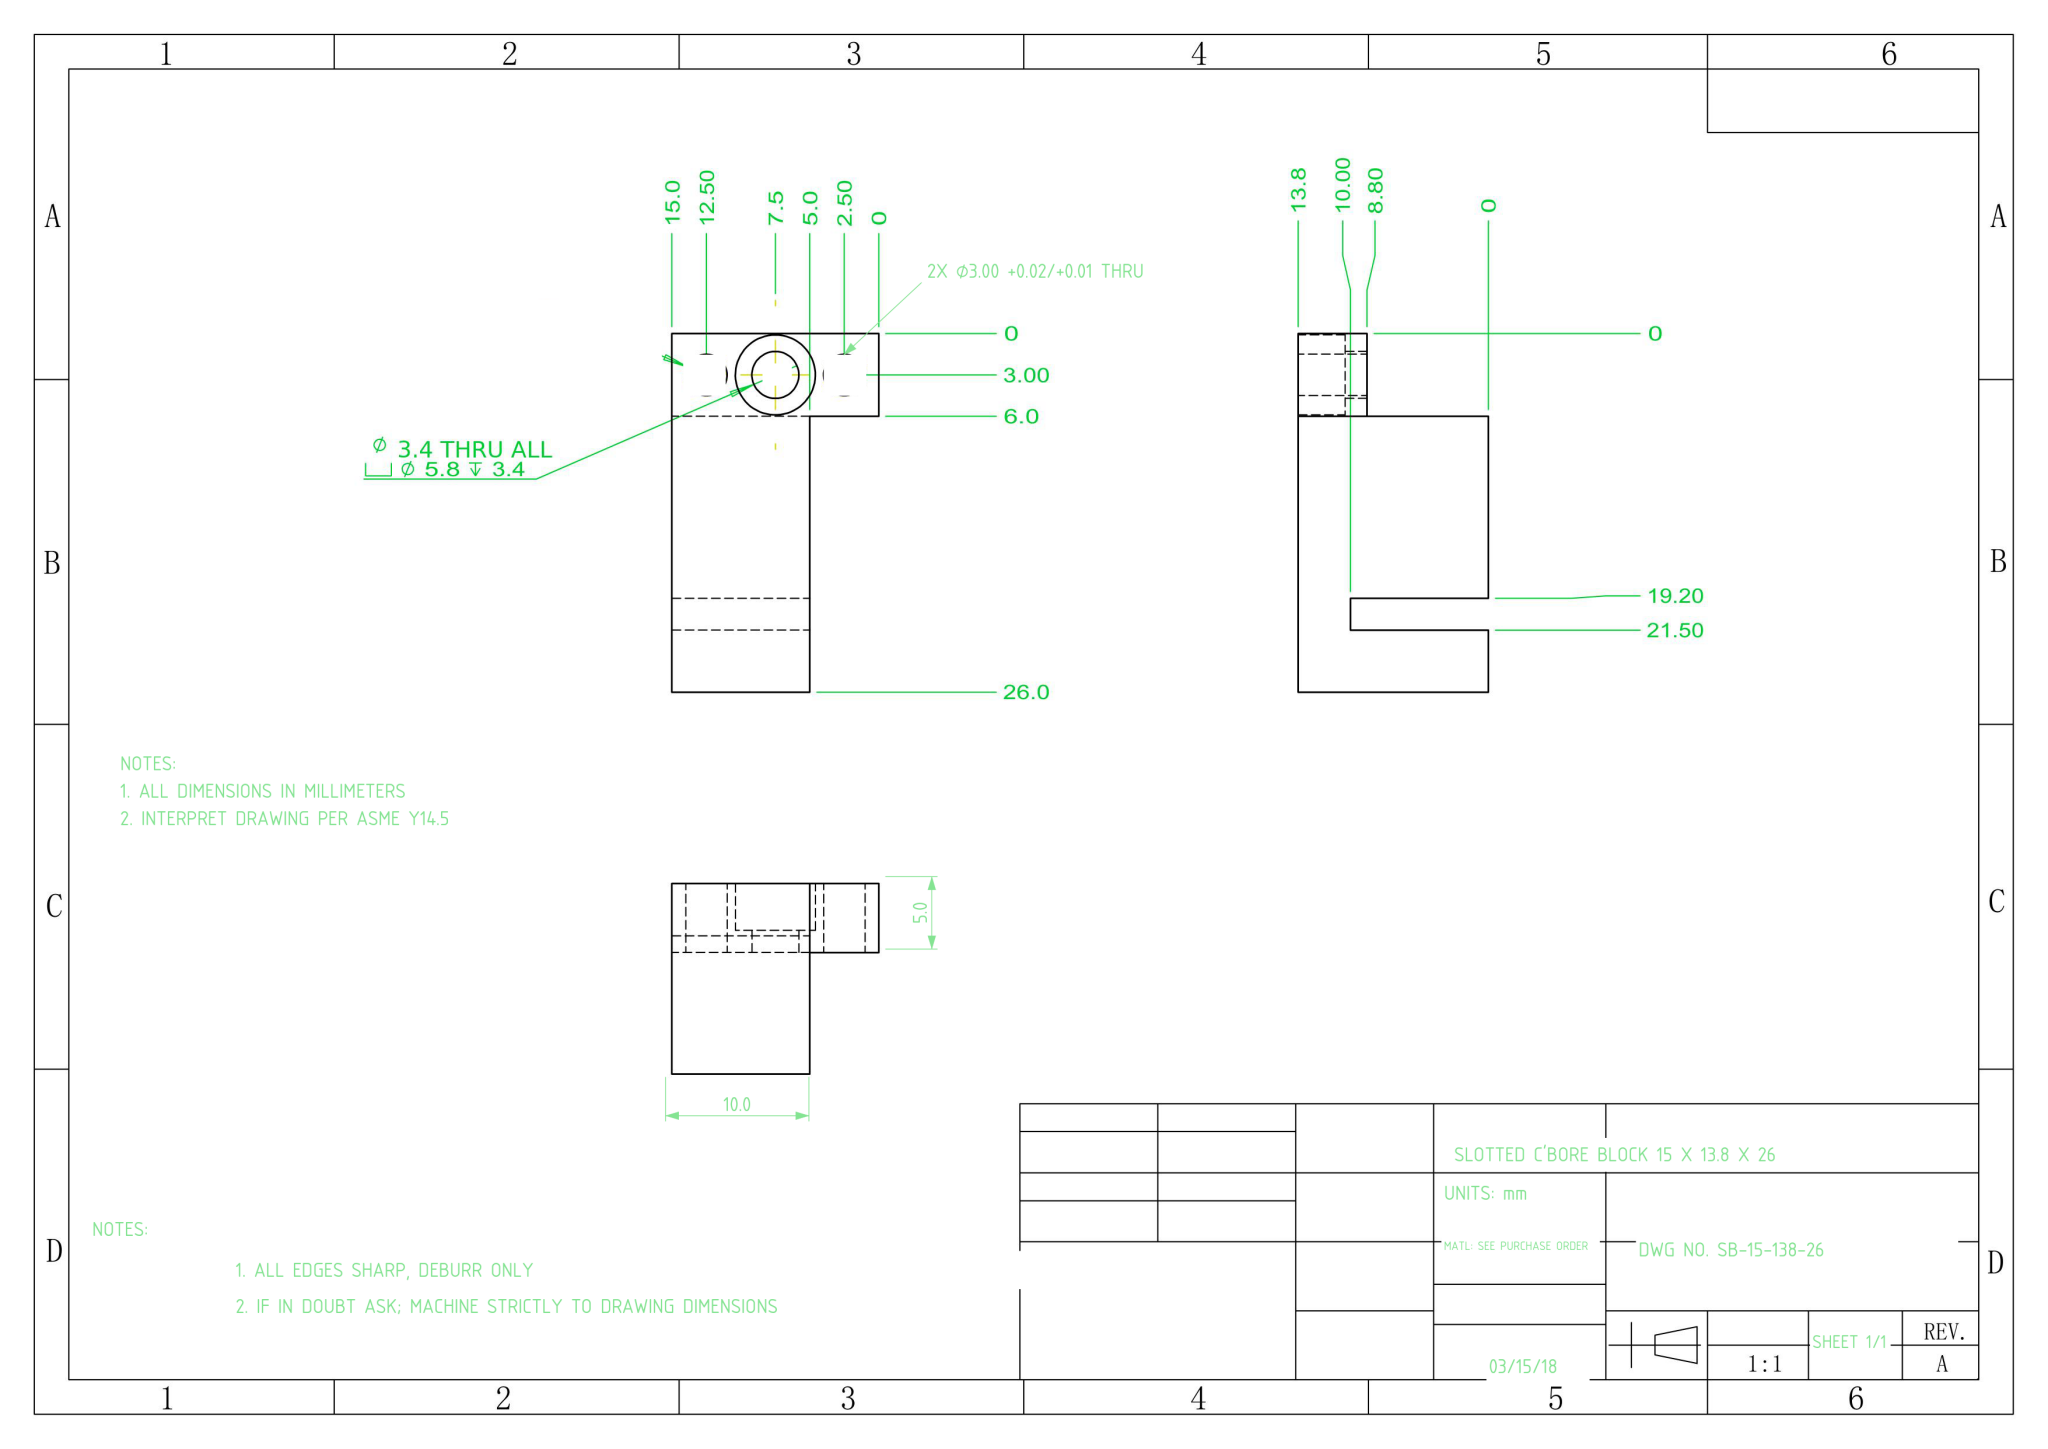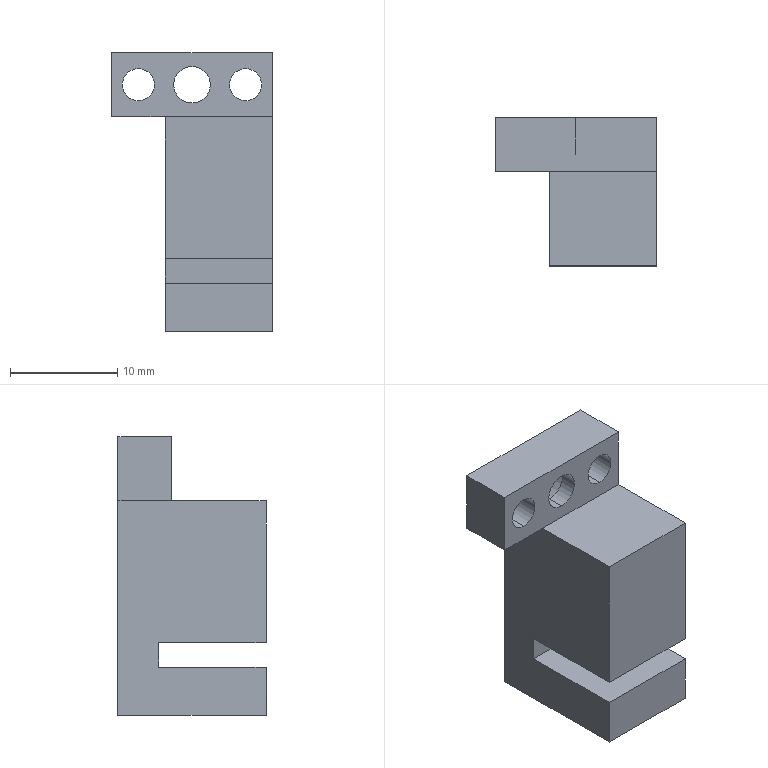Part | NX | mm | 1 solid | 23 faces | box 15 x 13.8 x 26 mm | volume 2805 mm3 | plane 15 | cylinder 8 | commonest cylinder face diameters 3 x4 5.8 x2 3.4 x2
STEP:
#1=COLOUR_RGB('',1.,0.4039,0.4431);
#2=FILL_AREA_STYLE_COLOUR('',#1);
#3=FILL_AREA_STYLE('',(#2));
#4=SURFACE_STYLE_FILL_AREA(#3);
#5=SURFACE_SIDE_STYLE('',(#4));
#6=SURFACE_STYLE_USAGE(.BOTH.,#5);
#7=PRESENTATION_STYLE_ASSIGNMENT((#6));
#8=CARTESIAN_POINT('',(2.5,-3.4,20.1));
#9=VERTEX_POINT('',#8);
#10=CARTESIAN_POINT('',(2.5,-3.4,25.9));
#11=VERTEX_POINT('',#10);
#12=CARTESIAN_POINT('',(2.5,-3.4,23.));
#13=DIRECTION('',(0.,1.,0.));
#14=DIRECTION('',(0.,0.,1.));
#15=AXIS2_PLACEMENT_3D('',#12,#13,#14);
#16=CIRCLE('',#15,2.9);
#17=EDGE_CURVE('',#9,#11,#16,.T.);
#18=ORIENTED_EDGE('',*,*,#17,.F.);
#19=CARTESIAN_POINT('',(2.5,0.,20.1));
#20=VERTEX_POINT('',#19);
#21=CARTESIAN_POINT('',(2.5,0.,20.1));
#22=DIRECTION('',(0.,1.,0.));
#23=VECTOR('',#22,1000.);
#24=LINE('',#21,#23);
#25=EDGE_CURVE('',#9,#20,#24,.T.);
#26=ORIENTED_EDGE('',*,*,#25,.T.);
#27=CARTESIAN_POINT('',(2.5,0.,25.9));
#28=VERTEX_POINT('',#27);
#29=CARTESIAN_POINT('',(2.5,0.,23.));
#30=DIRECTION('',(0.,1.,0.));
#31=DIRECTION('',(0.,0.,1.));
#32=AXIS2_PLACEMENT_3D('',#29,#30,#31);
#33=CIRCLE('',#32,2.9);
#34=EDGE_CURVE('',#20,#28,#33,.T.);
#35=ORIENTED_EDGE('',*,*,#34,.T.);
#36=CARTESIAN_POINT('',(2.5,0.,25.9));
#37=DIRECTION('',(0.,1.,0.));
#38=VECTOR('',#37,1000.);
#39=LINE('',#36,#38);
#40=EDGE_CURVE('',#11,#28,#39,.T.);
#41=ORIENTED_EDGE('',*,*,#40,.F.);
#42=EDGE_LOOP('',(#18,#26,#35,#41));
#43=FACE_OUTER_BOUND('',#42,.T.);
#44=CARTESIAN_POINT('',(2.5,0.,23.));
#45=DIRECTION('',(0.,1.,0.));
#46=DIRECTION('',(0.,0.,1.));
#47=AXIS2_PLACEMENT_3D('',#44,#45,#46);
#48=CYLINDRICAL_SURFACE('',#47,2.9);
#49=ADVANCED_FACE('',(#43),#48,.F.);
#50=CARTESIAN_POINT('',(2.5,-5.,21.3));
#51=VERTEX_POINT('',#50);
#52=CARTESIAN_POINT('',(2.5,-5.,24.7));
#53=VERTEX_POINT('',#52);
#54=CARTESIAN_POINT('',(2.5,-5.,23.));
#55=DIRECTION('',(0.,1.,0.));
#56=DIRECTION('',(0.,0.,1.));
#57=AXIS2_PLACEMENT_3D('',#54,#55,#56);
#58=CIRCLE('',#57,1.7);
#59=EDGE_CURVE('',#51,#53,#58,.T.);
#60=ORIENTED_EDGE('',*,*,#59,.F.);
#61=CARTESIAN_POINT('',(2.5,-3.4,21.3));
#62=VERTEX_POINT('',#61);
#63=CARTESIAN_POINT('',(2.5,0.,21.3));
#64=DIRECTION('',(0.,1.,0.));
#65=VECTOR('',#64,1000.);
#66=LINE('',#63,#65);
#67=EDGE_CURVE('',#51,#62,#66,.T.);
#68=ORIENTED_EDGE('',*,*,#67,.T.);
#69=CARTESIAN_POINT('',(2.5,-3.4,24.7));
#70=VERTEX_POINT('',#69);
#71=CARTESIAN_POINT('',(2.5,-3.4,23.));
#72=DIRECTION('',(0.,1.,0.));
#73=DIRECTION('',(0.,0.,1.));
#74=AXIS2_PLACEMENT_3D('',#71,#72,#73);
#75=CIRCLE('',#74,1.7);
#76=EDGE_CURVE('',#62,#70,#75,.T.);
#77=ORIENTED_EDGE('',*,*,#76,.T.);
#78=CARTESIAN_POINT('',(2.5,0.,24.7));
#79=DIRECTION('',(0.,1.,0.));
#80=VECTOR('',#79,1000.);
#81=LINE('',#78,#80);
#82=EDGE_CURVE('',#53,#70,#81,.T.);
#83=ORIENTED_EDGE('',*,*,#82,.F.);
#84=EDGE_LOOP('',(#60,#68,#77,#83));
#85=FACE_OUTER_BOUND('',#84,.T.);
#86=CARTESIAN_POINT('',(2.5,0.,23.));
#87=DIRECTION('',(0.,1.,0.));
#88=DIRECTION('',(0.,0.,1.));
#89=AXIS2_PLACEMENT_3D('',#86,#87,#88);
#90=CYLINDRICAL_SURFACE('',#89,1.7);
#91=ADVANCED_FACE('',(#85),#90,.F.);
#92=CARTESIAN_POINT('',(7.5,-5.,21.5));
#93=VERTEX_POINT('',#92);
#94=CARTESIAN_POINT('',(7.5,-5.,24.5));
#95=VERTEX_POINT('',#94);
#96=CARTESIAN_POINT('',(7.5,-5.,23.));
#97=DIRECTION('',(0.,1.,0.));
#98=DIRECTION('',(0.,0.,1.));
#99=AXIS2_PLACEMENT_3D('',#96,#97,#98);
#100=CIRCLE('',#99,1.5);
#101=EDGE_CURVE('',#93,#95,#100,.T.);
#102=ORIENTED_EDGE('',*,*,#101,.F.);
#103=CARTESIAN_POINT('',(7.5,0.,21.5));
#104=VERTEX_POINT('',#103);
#105=CARTESIAN_POINT('',(7.5,0.,21.5));
#106=DIRECTION('',(0.,1.,0.));
#107=VECTOR('',#106,1000.);
#108=LINE('',#105,#107);
#109=EDGE_CURVE('',#93,#104,#108,.T.);
#110=ORIENTED_EDGE('',*,*,#109,.T.);
#111=CARTESIAN_POINT('',(7.5,0.,24.5));
#112=VERTEX_POINT('',#111);
#113=CARTESIAN_POINT('',(7.5,0.,23.));
#114=DIRECTION('',(0.,1.,0.));
#115=DIRECTION('',(0.,0.,1.));
#116=AXIS2_PLACEMENT_3D('',#113,#114,#115);
#117=CIRCLE('',#116,1.5);
#118=EDGE_CURVE('',#104,#112,#117,.T.);
#119=ORIENTED_EDGE('',*,*,#118,.T.);
#120=CARTESIAN_POINT('',(7.5,0.,24.5));
#121=DIRECTION('',(0.,1.,0.));
#122=VECTOR('',#121,1000.);
#123=LINE('',#120,#122);
#124=EDGE_CURVE('',#95,#112,#123,.T.);
#125=ORIENTED_EDGE('',*,*,#124,.F.);
#126=EDGE_LOOP('',(#102,#110,#119,#125));
#127=FACE_OUTER_BOUND('',#126,.T.);
#128=CARTESIAN_POINT('',(7.5,0.,23.));
#129=DIRECTION('',(0.,1.,0.));
#130=DIRECTION('',(0.,0.,1.));
#131=AXIS2_PLACEMENT_3D('',#128,#129,#130);
#132=CYLINDRICAL_SURFACE('',#131,1.5);
#133=ADVANCED_FACE('',(#127),#132,.F.);
#134=CARTESIAN_POINT('',(-2.5,-5.,21.5));
#135=VERTEX_POINT('',#134);
#136=CARTESIAN_POINT('',(-2.5,-5.,24.5));
#137=VERTEX_POINT('',#136);
#138=CARTESIAN_POINT('',(-2.5,-5.,23.));
#139=DIRECTION('',(0.,1.,0.));
#140=DIRECTION('',(0.,0.,1.));
#141=AXIS2_PLACEMENT_3D('',#138,#139,#140);
#142=CIRCLE('',#141,1.5);
#143=EDGE_CURVE('',#135,#137,#142,.T.);
#144=ORIENTED_EDGE('',*,*,#143,.F.);
#145=CARTESIAN_POINT('',(-2.5,0.,21.5));
#146=VERTEX_POINT('',#145);
#147=CARTESIAN_POINT('',(-2.5,0.,21.5));
#148=DIRECTION('',(0.,1.,0.));
#149=VECTOR('',#148,1000.);
#150=LINE('',#147,#149);
#151=EDGE_CURVE('',#135,#146,#150,.T.);
#152=ORIENTED_EDGE('',*,*,#151,.T.);
#153=CARTESIAN_POINT('',(-2.5,0.,24.5));
#154=VERTEX_POINT('',#153);
#155=CARTESIAN_POINT('',(-2.5,0.,23.));
#156=DIRECTION('',(0.,1.,0.));
#157=DIRECTION('',(0.,0.,1.));
#158=AXIS2_PLACEMENT_3D('',#155,#156,#157);
#159=CIRCLE('',#158,1.5);
#160=EDGE_CURVE('',#146,#154,#159,.T.);
#161=ORIENTED_EDGE('',*,*,#160,.T.);
#162=CARTESIAN_POINT('',(-2.5,0.,24.5));
#163=DIRECTION('',(0.,1.,0.));
#164=VECTOR('',#163,1000.);
#165=LINE('',#162,#164);
#166=EDGE_CURVE('',#137,#154,#165,.T.);
#167=ORIENTED_EDGE('',*,*,#166,.F.);
#168=EDGE_LOOP('',(#144,#152,#161,#167));
#169=FACE_OUTER_BOUND('',#168,.T.);
#170=CARTESIAN_POINT('',(-2.5,0.,23.));
#171=DIRECTION('',(0.,1.,0.));
#172=DIRECTION('',(0.,0.,1.));
#173=AXIS2_PLACEMENT_3D('',#170,#171,#172);
#174=CYLINDRICAL_SURFACE('',#173,1.5);
#175=ADVANCED_FACE('',(#169),#174,.F.);
#176=CARTESIAN_POINT('',(10.,-13.8,4.5));
#177=VERTEX_POINT('',#176);
#178=CARTESIAN_POINT('',(10.,-13.8,0.));
#179=VERTEX_POINT('',#178);
#180=CARTESIAN_POINT('',(10.,-13.8,20.));
#181=DIRECTION('',(0.,0.,-1.));
#182=VECTOR('',#181,1000.);
#183=LINE('',#180,#182);
#184=EDGE_CURVE('',#177,#179,#183,.T.);
#185=ORIENTED_EDGE('',*,*,#184,.F.);
#186=CARTESIAN_POINT('',(0.,-13.8,4.5));
#187=VERTEX_POINT('',#186);
#188=CARTESIAN_POINT('',(10.,-13.8,4.5));
#189=DIRECTION('',(-1.,-0.,0.));
#190=VECTOR('',#189,1000.);
#191=LINE('',#188,#190);
#192=EDGE_CURVE('',#177,#187,#191,.T.);
#193=ORIENTED_EDGE('',*,*,#192,.T.);
#194=CARTESIAN_POINT('',(0.,-13.8,0.));
#195=VERTEX_POINT('',#194);
#196=CARTESIAN_POINT('',(0.,-13.8,20.));
#197=DIRECTION('',(0.,0.,-1.));
#198=VECTOR('',#197,1000.);
#199=LINE('',#196,#198);
#200=EDGE_CURVE('',#187,#195,#199,.T.);
#201=ORIENTED_EDGE('',*,*,#200,.T.);
#202=CARTESIAN_POINT('',(0.,-13.8,0.));
#203=DIRECTION('',(1.,0.,0.));
#204=VECTOR('',#203,1000.);
#205=LINE('',#202,#204);
#206=EDGE_CURVE('',#195,#179,#205,.T.);
#207=ORIENTED_EDGE('',*,*,#206,.T.);
#208=EDGE_LOOP('',(#185,#193,#201,#207));
#209=FACE_OUTER_BOUND('',#208,.T.);
#210=CARTESIAN_POINT('',(0.,-13.8,20.));
#211=DIRECTION('',(0.,1.,0.));
#212=DIRECTION('',(0.,0.,1.));
#213=AXIS2_PLACEMENT_3D('',#210,#211,#212);
#214=PLANE('',#213);
#215=ADVANCED_FACE('',(#209),#214,.F.);
#216=ORIENTED_EDGE('',*,*,#200,.F.);
#217=CARTESIAN_POINT('',(0.,-3.8,4.5));
#218=VERTEX_POINT('',#217);
#219=CARTESIAN_POINT('',(0.,-13.8,4.5));
#220=DIRECTION('',(0.,-1.,0.));
#221=VECTOR('',#220,1000.);
#222=LINE('',#219,#221);
#223=EDGE_CURVE('',#218,#187,#222,.T.);
#224=ORIENTED_EDGE('',*,*,#223,.F.);
#225=CARTESIAN_POINT('',(0.,-3.8,6.8));
#226=VERTEX_POINT('',#225);
#227=CARTESIAN_POINT('',(0.,-3.8,4.5));
#228=DIRECTION('',(0.,0.,-1.));
#229=VECTOR('',#228,1000.);
#230=LINE('',#227,#229);
#231=EDGE_CURVE('',#226,#218,#230,.T.);
#232=ORIENTED_EDGE('',*,*,#231,.F.);
#233=CARTESIAN_POINT('',(0.,-13.8,6.8));
#234=VERTEX_POINT('',#233);
#235=CARTESIAN_POINT('',(0.,-13.8,6.8));
#236=DIRECTION('',(-0.,1.,0.));
#237=VECTOR('',#236,1000.);
#238=LINE('',#235,#237);
#239=EDGE_CURVE('',#234,#226,#238,.T.);
#240=ORIENTED_EDGE('',*,*,#239,.F.);
#241=CARTESIAN_POINT('',(0.,-13.8,20.));
#242=VERTEX_POINT('',#241);
#243=CARTESIAN_POINT('',(0.,-13.8,20.));
#244=DIRECTION('',(0.,0.,-1.));
#245=VECTOR('',#244,1000.);
#246=LINE('',#243,#245);
#247=EDGE_CURVE('',#242,#234,#246,.T.);
#248=ORIENTED_EDGE('',*,*,#247,.F.);
#249=CARTESIAN_POINT('',(0.,-5.,20.));
#250=VERTEX_POINT('',#249);
#251=CARTESIAN_POINT('',(0.,0.,20.));
#252=DIRECTION('',(0.,-1.,0.));
#253=VECTOR('',#252,1000.);
#254=LINE('',#251,#253);
#255=EDGE_CURVE('',#250,#242,#254,.T.);
#256=ORIENTED_EDGE('',*,*,#255,.F.);
#257=CARTESIAN_POINT('',(0.,0.,20.));
#258=VERTEX_POINT('',#257);
#259=CARTESIAN_POINT('',(0.,0.,20.));
#260=DIRECTION('',(0.,-1.,0.));
#261=VECTOR('',#260,1000.);
#262=LINE('',#259,#261);
#263=EDGE_CURVE('',#258,#250,#262,.T.);
#264=ORIENTED_EDGE('',*,*,#263,.F.);
#265=CARTESIAN_POINT('',(0.,0.,0.));
#266=VERTEX_POINT('',#265);
#267=CARTESIAN_POINT('',(0.,0.,20.));
#268=DIRECTION('',(0.,0.,-1.));
#269=VECTOR('',#268,1000.);
#270=LINE('',#267,#269);
#271=EDGE_CURVE('',#258,#266,#270,.T.);
#272=ORIENTED_EDGE('',*,*,#271,.T.);
#273=CARTESIAN_POINT('',(0.,0.,0.));
#274=DIRECTION('',(0.,-1.,0.));
#275=VECTOR('',#274,1000.);
#276=LINE('',#273,#275);
#277=EDGE_CURVE('',#266,#195,#276,.T.);
#278=ORIENTED_EDGE('',*,*,#277,.T.);
#279=EDGE_LOOP('',(#216,#224,#232,#240,#248,#256,#264,#272,#278));
#280=FACE_OUTER_BOUND('',#279,.T.);
#281=CARTESIAN_POINT('',(0.,0.,20.));
#282=DIRECTION('',(1.,0.,0.));
#283=DIRECTION('',(-0.,1.,0.));
#284=AXIS2_PLACEMENT_3D('',#281,#282,#283);
#285=PLANE('',#284);
#286=ADVANCED_FACE('',(#280),#285,.F.);
#287=ORIENTED_EDGE('',*,*,#247,.T.);
#288=CARTESIAN_POINT('',(10.,-13.8,6.8));
#289=VERTEX_POINT('',#288);
#290=CARTESIAN_POINT('',(10.,-13.8,6.8));
#291=DIRECTION('',(-1.,-0.,0.));
#292=VECTOR('',#291,1000.);
#293=LINE('',#290,#292);
#294=EDGE_CURVE('',#289,#234,#293,.T.);
#295=ORIENTED_EDGE('',*,*,#294,.F.);
#296=CARTESIAN_POINT('',(10.,-13.8,20.));
#297=VERTEX_POINT('',#296);
#298=CARTESIAN_POINT('',(10.,-13.8,20.));
#299=DIRECTION('',(0.,0.,-1.));
#300=VECTOR('',#299,1000.);
#301=LINE('',#298,#300);
#302=EDGE_CURVE('',#297,#289,#301,.T.);
#303=ORIENTED_EDGE('',*,*,#302,.F.);
#304=CARTESIAN_POINT('',(0.,-13.8,20.));
#305=DIRECTION('',(1.,0.,0.));
#306=VECTOR('',#305,1000.);
#307=LINE('',#304,#306);
#308=EDGE_CURVE('',#242,#297,#307,.T.);
#309=ORIENTED_EDGE('',*,*,#308,.F.);
#310=EDGE_LOOP('',(#287,#295,#303,#309));
#311=FACE_OUTER_BOUND('',#310,.T.);
#312=CARTESIAN_POINT('',(0.,-13.8,20.));
#313=DIRECTION('',(0.,1.,0.));
#314=DIRECTION('',(0.,0.,1.));
#315=AXIS2_PLACEMENT_3D('',#312,#313,#314);
#316=PLANE('',#315);
#317=ADVANCED_FACE('',(#311),#316,.F.);
#318=CARTESIAN_POINT('',(10.,-3.8,6.8));
#319=VERTEX_POINT('',#318);
#320=CARTESIAN_POINT('',(10.,-3.8,4.5));
#321=VERTEX_POINT('',#320);
#322=CARTESIAN_POINT('',(10.,-3.8,4.5));
#323=DIRECTION('',(0.,0.,-1.));
#324=VECTOR('',#323,1000.);
#325=LINE('',#322,#324);
#326=EDGE_CURVE('',#319,#321,#325,.T.);
#327=ORIENTED_EDGE('',*,*,#326,.T.);
#328=CARTESIAN_POINT('',(10.,-13.8,4.5));
#329=DIRECTION('',(0.,-1.,0.));
#330=VECTOR('',#329,1000.);
#331=LINE('',#328,#330);
#332=EDGE_CURVE('',#321,#177,#331,.T.);
#333=ORIENTED_EDGE('',*,*,#332,.T.);
#334=ORIENTED_EDGE('',*,*,#184,.T.);
#335=CARTESIAN_POINT('',(10.,0.,0.));
#336=VERTEX_POINT('',#335);
#337=CARTESIAN_POINT('',(10.,0.,0.));
#338=DIRECTION('',(-0.,1.,0.));
#339=VECTOR('',#338,1000.);
#340=LINE('',#337,#339);
#341=EDGE_CURVE('',#179,#336,#340,.T.);
#342=ORIENTED_EDGE('',*,*,#341,.T.);
#343=CARTESIAN_POINT('',(10.,0.,26.));
#344=VERTEX_POINT('',#343);
#345=CARTESIAN_POINT('',(10.,0.,20.));
#346=DIRECTION('',(0.,0.,-1.));
#347=VECTOR('',#346,1000.);
#348=LINE('',#345,#347);
#349=EDGE_CURVE('',#344,#336,#348,.T.);
#350=ORIENTED_EDGE('',*,*,#349,.F.);
#351=CARTESIAN_POINT('',(10.,-5.,26.));
#352=VERTEX_POINT('',#351);
#353=CARTESIAN_POINT('',(10.,0.,26.));
#354=DIRECTION('',(0.,1.,0.));
#355=VECTOR('',#354,1000.);
#356=LINE('',#353,#355);
#357=EDGE_CURVE('',#352,#344,#356,.T.);
#358=ORIENTED_EDGE('',*,*,#357,.F.);
#359=CARTESIAN_POINT('',(10.,-5.,20.));
#360=VERTEX_POINT('',#359);
#361=CARTESIAN_POINT('',(10.,-5.,26.));
#362=DIRECTION('',(0.,0.,-1.));
#363=VECTOR('',#362,1000.);
#364=LINE('',#361,#363);
#365=EDGE_CURVE('',#352,#360,#364,.T.);
#366=ORIENTED_EDGE('',*,*,#365,.T.);
#367=CARTESIAN_POINT('',(10.,0.,20.));
#368=DIRECTION('',(-0.,1.,0.));
#369=VECTOR('',#368,1000.);
#370=LINE('',#367,#369);
#371=EDGE_CURVE('',#297,#360,#370,.T.);
#372=ORIENTED_EDGE('',*,*,#371,.F.);
#373=ORIENTED_EDGE('',*,*,#302,.T.);
#374=CARTESIAN_POINT('',(10.,-13.8,6.8));
#375=DIRECTION('',(-0.,1.,0.));
#376=VECTOR('',#375,1000.);
#377=LINE('',#374,#376);
#378=EDGE_CURVE('',#289,#319,#377,.T.);
#379=ORIENTED_EDGE('',*,*,#378,.T.);
#380=EDGE_LOOP('',(#327,#333,#334,#342,#350,#358,#366,#372,#373,#379));
#381=FACE_OUTER_BOUND('',#380,.T.);
#382=CARTESIAN_POINT('',(10.,0.,20.));
#383=DIRECTION('',(-1.,-0.,0.));
#384=DIRECTION('',(0.,-1.,0.));
#385=AXIS2_PLACEMENT_3D('',#382,#383,#384);
#386=PLANE('',#385);
#387=ADVANCED_FACE('',(#381),#386,.F.);
#388=CARTESIAN_POINT('',(2.5,0.,23.));
#389=DIRECTION('',(0.,1.,0.));
#390=DIRECTION('',(0.,0.,1.));
#391=AXIS2_PLACEMENT_3D('',#388,#389,#390);
#392=CIRCLE('',#391,2.9);
#393=EDGE_CURVE('',#28,#20,#392,.T.);
#394=ORIENTED_EDGE('',*,*,#393,.F.);
#395=ORIENTED_EDGE('',*,*,#34,.F.);
#396=EDGE_LOOP('',(#394,#395));
#397=FACE_BOUND('',#396,.T.);
#398=CARTESIAN_POINT('',(7.5,0.,23.));
#399=DIRECTION('',(0.,1.,0.));
#400=DIRECTION('',(0.,0.,1.));
#401=AXIS2_PLACEMENT_3D('',#398,#399,#400);
#402=CIRCLE('',#401,1.5);
#403=EDGE_CURVE('',#112,#104,#402,.T.);
#404=ORIENTED_EDGE('',*,*,#403,.F.);
#405=ORIENTED_EDGE('',*,*,#118,.F.);
#406=EDGE_LOOP('',(#404,#405));
#407=FACE_BOUND('',#406,.T.);
#408=CARTESIAN_POINT('',(-2.5,0.,23.));
#409=DIRECTION('',(0.,1.,0.));
#410=DIRECTION('',(0.,0.,1.));
#411=AXIS2_PLACEMENT_3D('',#408,#409,#410);
#412=CIRCLE('',#411,1.5);
#413=EDGE_CURVE('',#154,#146,#412,.T.);
#414=ORIENTED_EDGE('',*,*,#413,.F.);
#415=ORIENTED_EDGE('',*,*,#160,.F.);
#416=EDGE_LOOP('',(#414,#415));
#417=FACE_BOUND('',#416,.T.);
#418=CARTESIAN_POINT('',(0.,0.,0.));
#419=DIRECTION('',(-1.,0.,0.));
#420=VECTOR('',#419,1000.);
#421=LINE('',#418,#420);
#422=EDGE_CURVE('',#336,#266,#421,.T.);
#423=ORIENTED_EDGE('',*,*,#422,.T.);
#424=ORIENTED_EDGE('',*,*,#271,.F.);
#425=CARTESIAN_POINT('',(-5.,-0.,20.));
#426=VERTEX_POINT('',#425);
#427=CARTESIAN_POINT('',(-5.,-0.,20.));
#428=DIRECTION('',(1.,0.,0.));
#429=VECTOR('',#428,1000.);
#430=LINE('',#427,#429);
#431=EDGE_CURVE('',#426,#258,#430,.T.);
#432=ORIENTED_EDGE('',*,*,#431,.F.);
#433=CARTESIAN_POINT('',(-5.,0.,26.));
#434=VERTEX_POINT('',#433);
#435=CARTESIAN_POINT('',(-5.,0.,26.));
#436=DIRECTION('',(0.,-0.,-1.));
#437=VECTOR('',#436,1000.);
#438=LINE('',#435,#437);
#439=EDGE_CURVE('',#434,#426,#438,.T.);
#440=ORIENTED_EDGE('',*,*,#439,.F.);
#441=CARTESIAN_POINT('',(0.,0.,26.));
#442=DIRECTION('',(-1.,0.,0.));
#443=VECTOR('',#442,1000.);
#444=LINE('',#441,#443);
#445=EDGE_CURVE('',#344,#434,#444,.T.);
#446=ORIENTED_EDGE('',*,*,#445,.F.);
#447=ORIENTED_EDGE('',*,*,#349,.T.);
#448=EDGE_LOOP('',(#423,#424,#432,#440,#446,#447));
#449=FACE_OUTER_BOUND('',#448,.T.);
#450=CARTESIAN_POINT('',(0.,0.,20.));
#451=DIRECTION('',(0.,-1.,0.));
#452=DIRECTION('',(0.,0.,-1.));
#453=AXIS2_PLACEMENT_3D('',#450,#451,#452);
#454=PLANE('',#453);
#455=ADVANCED_FACE('',(#397,#407,#417,#449),#454,.F.);
#456=CARTESIAN_POINT('',(0.,-5.,20.));
#457=DIRECTION('',(1.,0.,0.));
#458=VECTOR('',#457,1000.);
#459=LINE('',#456,#458);
#460=EDGE_CURVE('',#250,#360,#459,.T.);
#461=ORIENTED_EDGE('',*,*,#460,.F.);
#462=ORIENTED_EDGE('',*,*,#255,.T.);
#463=ORIENTED_EDGE('',*,*,#308,.T.);
#464=ORIENTED_EDGE('',*,*,#371,.T.);
#465=EDGE_LOOP('',(#461,#462,#463,#464));
#466=FACE_OUTER_BOUND('',#465,.T.);
#467=CARTESIAN_POINT('',(0.,0.,20.));
#468=DIRECTION('',(0.,0.,1.));
#469=DIRECTION('',(1.,0.,0.));
#470=AXIS2_PLACEMENT_3D('',#467,#468,#469);
#471=PLANE('',#470);
#472=ADVANCED_FACE('',(#466),#471,.T.);
#473=ORIENTED_EDGE('',*,*,#277,.F.);
#474=ORIENTED_EDGE('',*,*,#422,.F.);
#475=ORIENTED_EDGE('',*,*,#341,.F.);
#476=ORIENTED_EDGE('',*,*,#206,.F.);
#477=EDGE_LOOP('',(#473,#474,#475,#476));
#478=FACE_OUTER_BOUND('',#477,.T.);
#479=CARTESIAN_POINT('',(0.,0.,0.));
#480=DIRECTION('',(0.,0.,1.));
#481=DIRECTION('',(1.,0.,0.));
#482=AXIS2_PLACEMENT_3D('',#479,#480,#481);
#483=PLANE('',#482);
#484=ADVANCED_FACE('',(#478),#483,.F.);
#485=CARTESIAN_POINT('',(2.5,-5.,23.));
#486=DIRECTION('',(0.,1.,0.));
#487=DIRECTION('',(0.,0.,1.));
#488=AXIS2_PLACEMENT_3D('',#485,#486,#487);
#489=CIRCLE('',#488,1.7);
#490=EDGE_CURVE('',#53,#51,#489,.T.);
#491=ORIENTED_EDGE('',*,*,#490,.T.);
#492=ORIENTED_EDGE('',*,*,#59,.T.);
#493=EDGE_LOOP('',(#491,#492));
#494=FACE_BOUND('',#493,.T.);
#495=CARTESIAN_POINT('',(7.5,-5.,23.));
#496=DIRECTION('',(0.,1.,0.));
#497=DIRECTION('',(0.,0.,1.));
#498=AXIS2_PLACEMENT_3D('',#495,#496,#497);
#499=CIRCLE('',#498,1.5);
#500=EDGE_CURVE('',#95,#93,#499,.T.);
#501=ORIENTED_EDGE('',*,*,#500,.T.);
#502=ORIENTED_EDGE('',*,*,#101,.T.);
#503=EDGE_LOOP('',(#501,#502));
#504=FACE_BOUND('',#503,.T.);
#505=CARTESIAN_POINT('',(-2.5,-5.,23.));
#506=DIRECTION('',(0.,1.,0.));
#507=DIRECTION('',(0.,0.,1.));
#508=AXIS2_PLACEMENT_3D('',#505,#506,#507);
#509=CIRCLE('',#508,1.5);
#510=EDGE_CURVE('',#137,#135,#509,.T.);
#511=ORIENTED_EDGE('',*,*,#510,.T.);
#512=ORIENTED_EDGE('',*,*,#143,.T.);
#513=EDGE_LOOP('',(#511,#512));
#514=FACE_BOUND('',#513,.T.);
#515=ORIENTED_EDGE('',*,*,#460,.T.);
#516=ORIENTED_EDGE('',*,*,#365,.F.);
#517=CARTESIAN_POINT('',(-5.,-5.,26.));
#518=VERTEX_POINT('',#517);
#519=CARTESIAN_POINT('',(0.,-5.,26.));
#520=DIRECTION('',(1.,0.,0.));
#521=VECTOR('',#520,1000.);
#522=LINE('',#519,#521);
#523=EDGE_CURVE('',#518,#352,#522,.T.);
#524=ORIENTED_EDGE('',*,*,#523,.F.);
#525=CARTESIAN_POINT('',(-5.,-5.,20.));
#526=VERTEX_POINT('',#525);
#527=CARTESIAN_POINT('',(-5.,-5.,26.));
#528=DIRECTION('',(-0.,0.,1.));
#529=VECTOR('',#528,1000.);
#530=LINE('',#527,#529);
#531=EDGE_CURVE('',#526,#518,#530,.T.);
#532=ORIENTED_EDGE('',*,*,#531,.F.);
#533=CARTESIAN_POINT('',(-5.,-5.,20.));
#534=DIRECTION('',(1.,0.,0.));
#535=VECTOR('',#534,1000.);
#536=LINE('',#533,#535);
#537=EDGE_CURVE('',#526,#250,#536,.T.);
#538=ORIENTED_EDGE('',*,*,#537,.T.);
#539=EDGE_LOOP('',(#515,#516,#524,#532,#538));
#540=FACE_OUTER_BOUND('',#539,.T.);
#541=CARTESIAN_POINT('',(0.,-5.,26.));
#542=DIRECTION('',(0.,1.,0.));
#543=DIRECTION('',(0.,0.,1.));
#544=AXIS2_PLACEMENT_3D('',#541,#542,#543);
#545=PLANE('',#544);
#546=ADVANCED_FACE('',(#494,#504,#514,#540),#545,.F.);
#547=ORIENTED_EDGE('',*,*,#445,.T.);
#548=CARTESIAN_POINT('',(-5.,0.,26.));
#549=DIRECTION('',(-0.,1.,0.));
#550=VECTOR('',#549,1000.);
#551=LINE('',#548,#550);
#552=EDGE_CURVE('',#518,#434,#551,.T.);
#553=ORIENTED_EDGE('',*,*,#552,.F.);
#554=ORIENTED_EDGE('',*,*,#523,.T.);
#555=ORIENTED_EDGE('',*,*,#357,.T.);
#556=EDGE_LOOP('',(#547,#553,#554,#555));
#557=FACE_OUTER_BOUND('',#556,.T.);
#558=CARTESIAN_POINT('',(0.,0.,26.));
#559=DIRECTION('',(0.,0.,1.));
#560=DIRECTION('',(1.,0.,0.));
#561=AXIS2_PLACEMENT_3D('',#558,#559,#560);
#562=PLANE('',#561);
#563=ADVANCED_FACE('',(#557),#562,.T.);
#564=ORIENTED_EDGE('',*,*,#263,.T.);
#565=ORIENTED_EDGE('',*,*,#537,.F.);
#566=CARTESIAN_POINT('',(-5.,-0.,20.));
#567=DIRECTION('',(0.,-1.,0.));
#568=VECTOR('',#567,1000.);
#569=LINE('',#566,#568);
#570=EDGE_CURVE('',#426,#526,#569,.T.);
#571=ORIENTED_EDGE('',*,*,#570,.F.);
#572=ORIENTED_EDGE('',*,*,#431,.T.);
#573=EDGE_LOOP('',(#564,#565,#571,#572));
#574=FACE_OUTER_BOUND('',#573,.T.);
#575=CARTESIAN_POINT('',(-5.,-0.,20.));
#576=DIRECTION('',(0.,0.,1.));
#577=DIRECTION('',(1.,0.,0.));
#578=AXIS2_PLACEMENT_3D('',#575,#576,#577);
#579=PLANE('',#578);
#580=ADVANCED_FACE('',(#574),#579,.F.);
#581=ORIENTED_EDGE('',*,*,#552,.T.);
#582=ORIENTED_EDGE('',*,*,#439,.T.);
#583=ORIENTED_EDGE('',*,*,#570,.T.);
#584=ORIENTED_EDGE('',*,*,#531,.T.);
#585=EDGE_LOOP('',(#581,#582,#583,#584));
#586=FACE_OUTER_BOUND('',#585,.T.);
#587=CARTESIAN_POINT('',(-5.,-0.,0.));
#588=DIRECTION('',(1.,0.,-0.));
#589=DIRECTION('',(-0.,1.,0.));
#590=AXIS2_PLACEMENT_3D('',#587,#588,#589);
#591=PLANE('',#590);
#592=ADVANCED_FACE('',(#586),#591,.F.);
#593=ORIENTED_EDGE('',*,*,#223,.T.);
#594=ORIENTED_EDGE('',*,*,#192,.F.);
#595=ORIENTED_EDGE('',*,*,#332,.F.);
#596=CARTESIAN_POINT('',(10.,-3.8,4.5));
#597=DIRECTION('',(-1.,-0.,0.));
#598=VECTOR('',#597,1000.);
#599=LINE('',#596,#598);
#600=EDGE_CURVE('',#321,#218,#599,.T.);
#601=ORIENTED_EDGE('',*,*,#600,.T.);
#602=EDGE_LOOP('',(#593,#594,#595,#601));
#603=FACE_OUTER_BOUND('',#602,.T.);
#604=CARTESIAN_POINT('',(10.,-13.8,4.5));
#605=DIRECTION('',(0.,-0.,-1.));
#606=DIRECTION('',(0.,1.,-0.));
#607=AXIS2_PLACEMENT_3D('',#604,#605,#606);
#608=PLANE('',#607);
#609=ADVANCED_FACE('',(#603),#608,.F.);
#610=ORIENTED_EDGE('',*,*,#231,.T.);
#611=ORIENTED_EDGE('',*,*,#600,.F.);
#612=ORIENTED_EDGE('',*,*,#326,.F.);
#613=CARTESIAN_POINT('',(10.,-3.8,6.8));
#614=DIRECTION('',(-1.,-0.,0.));
#615=VECTOR('',#614,1000.);
#616=LINE('',#613,#615);
#617=EDGE_CURVE('',#319,#226,#616,.T.);
#618=ORIENTED_EDGE('',*,*,#617,.T.);
#619=EDGE_LOOP('',(#610,#611,#612,#618));
#620=FACE_OUTER_BOUND('',#619,.T.);
#621=CARTESIAN_POINT('',(10.,-3.8,4.5));
#622=DIRECTION('',(-0.,1.,0.));
#623=DIRECTION('',(-1.,-0.,0.));
#624=AXIS2_PLACEMENT_3D('',#621,#622,#623);
#625=PLANE('',#624);
#626=ADVANCED_FACE('',(#620),#625,.F.);
#627=ORIENTED_EDGE('',*,*,#239,.T.);
#628=ORIENTED_EDGE('',*,*,#617,.F.);
#629=ORIENTED_EDGE('',*,*,#378,.F.);
#630=ORIENTED_EDGE('',*,*,#294,.T.);
#631=EDGE_LOOP('',(#627,#628,#629,#630));
#632=FACE_OUTER_BOUND('',#631,.T.);
#633=CARTESIAN_POINT('',(10.,-13.8,6.8));
#634=DIRECTION('',(0.,0.,1.));
#635=DIRECTION('',(1.,0.,0.));
#636=AXIS2_PLACEMENT_3D('',#633,#634,#635);
#637=PLANE('',#636);
#638=ADVANCED_FACE('',(#632),#637,.F.);
#639=ORIENTED_EDGE('',*,*,#151,.F.);
#640=ORIENTED_EDGE('',*,*,#510,.F.);
#641=ORIENTED_EDGE('',*,*,#166,.T.);
#642=ORIENTED_EDGE('',*,*,#413,.T.);
#643=EDGE_LOOP('',(#639,#640,#641,#642));
#644=FACE_OUTER_BOUND('',#643,.T.);
#645=CARTESIAN_POINT('',(-2.5,0.,23.));
#646=DIRECTION('',(0.,1.,0.));
#647=DIRECTION('',(0.,0.,1.));
#648=AXIS2_PLACEMENT_3D('',#645,#646,#647);
#649=CYLINDRICAL_SURFACE('',#648,1.5);
#650=ADVANCED_FACE('',(#644),#649,.F.);
#651=ORIENTED_EDGE('',*,*,#109,.F.);
#652=ORIENTED_EDGE('',*,*,#500,.F.);
#653=ORIENTED_EDGE('',*,*,#124,.T.);
#654=ORIENTED_EDGE('',*,*,#403,.T.);
#655=EDGE_LOOP('',(#651,#652,#653,#654));
#656=FACE_OUTER_BOUND('',#655,.T.);
#657=CARTESIAN_POINT('',(7.5,0.,23.));
#658=DIRECTION('',(0.,1.,0.));
#659=DIRECTION('',(0.,0.,1.));
#660=AXIS2_PLACEMENT_3D('',#657,#658,#659);
#661=CYLINDRICAL_SURFACE('',#660,1.5);
#662=ADVANCED_FACE('',(#656),#661,.F.);
#663=ORIENTED_EDGE('',*,*,#67,.F.);
#664=ORIENTED_EDGE('',*,*,#490,.F.);
#665=ORIENTED_EDGE('',*,*,#82,.T.);
#666=CARTESIAN_POINT('',(2.5,-3.4,23.));
#667=DIRECTION('',(0.,1.,0.));
#668=DIRECTION('',(0.,0.,1.));
#669=AXIS2_PLACEMENT_3D('',#666,#667,#668);
#670=CIRCLE('',#669,1.7);
#671=EDGE_CURVE('',#70,#62,#670,.T.);
#672=ORIENTED_EDGE('',*,*,#671,.T.);
#673=EDGE_LOOP('',(#663,#664,#665,#672));
#674=FACE_OUTER_BOUND('',#673,.T.);
#675=CARTESIAN_POINT('',(2.5,0.,23.));
#676=DIRECTION('',(0.,1.,0.));
#677=DIRECTION('',(0.,0.,1.));
#678=AXIS2_PLACEMENT_3D('',#675,#676,#677);
#679=CYLINDRICAL_SURFACE('',#678,1.7);
#680=ADVANCED_FACE('',(#674),#679,.F.);
#681=ORIENTED_EDGE('',*,*,#671,.F.);
#682=ORIENTED_EDGE('',*,*,#76,.F.);
#683=EDGE_LOOP('',(#681,#682));
#684=FACE_BOUND('',#683,.T.);
#685=CARTESIAN_POINT('',(2.5,-3.4,23.));
#686=DIRECTION('',(0.,1.,0.));
#687=DIRECTION('',(0.,0.,1.));
#688=AXIS2_PLACEMENT_3D('',#685,#686,#687);
#689=CIRCLE('',#688,2.9);
#690=EDGE_CURVE('',#11,#9,#689,.T.);
#691=ORIENTED_EDGE('',*,*,#690,.T.);
#692=ORIENTED_EDGE('',*,*,#17,.T.);
#693=EDGE_LOOP('',(#691,#692));
#694=FACE_OUTER_BOUND('',#693,.T.);
#695=CARTESIAN_POINT('',(4.2,-3.4,23.));
#696=DIRECTION('',(0.,-1.,0.));
#697=DIRECTION('',(0.,0.,-1.));
#698=AXIS2_PLACEMENT_3D('',#695,#696,#697);
#699=PLANE('',#698);
#700=ADVANCED_FACE('',(#684,#694),#699,.F.);
#701=ORIENTED_EDGE('',*,*,#25,.F.);
#702=ORIENTED_EDGE('',*,*,#690,.F.);
#703=ORIENTED_EDGE('',*,*,#40,.T.);
#704=ORIENTED_EDGE('',*,*,#393,.T.);
#705=EDGE_LOOP('',(#701,#702,#703,#704));
#706=FACE_OUTER_BOUND('',#705,.T.);
#707=CARTESIAN_POINT('',(2.5,0.,23.));
#708=DIRECTION('',(0.,1.,0.));
#709=DIRECTION('',(0.,0.,1.));
#710=AXIS2_PLACEMENT_3D('',#707,#708,#709);
#711=CYLINDRICAL_SURFACE('',#710,2.9);
#712=ADVANCED_FACE('',(#706),#711,.F.);
#713=CLOSED_SHELL('',(#49,#91,#133,#175,#215,#286,#317,#387,#455,#472,#484,#546,#563,#580,#592,#609,#626,#638,#650,#662,#680,#700,#712));
#714=MANIFOLD_SOLID_BREP('',#713);
#715=CARTESIAN_POINT('',(0.,0.,0.));
#716=DIRECTION('',(0.,0.,1.));
#717=DIRECTION('',(1.,0.,0.));
#718=AXIS2_PLACEMENT_3D('',#715,#716,#717);
#719=(LENGTH_UNIT()NAMED_UNIT(*)SI_UNIT(.MILLI.,.METRE.));
#720=UNCERTAINTY_MEASURE_WITH_UNIT(LENGTH_MEASURE(0.00001),#719,'','');
#721=(NAMED_UNIT(*)PLANE_ANGLE_UNIT()SI_UNIT($,.RADIAN.));
#722=(NAMED_UNIT(*)SI_UNIT($,.STERADIAN.)SOLID_ANGLE_UNIT());
#723=(GEOMETRIC_REPRESENTATION_CONTEXT(3)GLOBAL_UNCERTAINTY_ASSIGNED_CONTEXT((#720))GLOBAL_UNIT_ASSIGNED_CONTEXT((#719,#721,#722))REPRESENTATION_CONTEXT('',''));
#724=ADVANCED_BREP_SHAPE_REPRESENTATION('',(#714,#718),#723);
#725=STYLED_ITEM('',(#7),#724);
#726=PRESENTATION_LAYER_ASSIGNMENT('','',(#725));
#727=COLOUR_RGB('',1.,0.4039,0.4431);
#728=FILL_AREA_STYLE_COLOUR('',#727);
#729=FILL_AREA_STYLE('',(#728));
#730=SURFACE_STYLE_FILL_AREA(#729);
#731=SURFACE_SIDE_STYLE('',(#730));
#732=SURFACE_STYLE_USAGE(.BOTH.,#731);
#733=PRESENTATION_STYLE_ASSIGNMENT((#732));
#734=STYLED_ITEM('',(#733),#714);
#735=(LENGTH_UNIT()NAMED_UNIT(*)SI_UNIT(.MILLI.,.METRE.));
#736=UNCERTAINTY_MEASURE_WITH_UNIT(LENGTH_MEASURE(0.00001),#735,'','');
#737=(NAMED_UNIT(*)PLANE_ANGLE_UNIT()SI_UNIT($,.RADIAN.));
#738=(NAMED_UNIT(*)SI_UNIT($,.STERADIAN.)SOLID_ANGLE_UNIT());
#739=(GEOMETRIC_REPRESENTATION_CONTEXT(3)GLOBAL_UNCERTAINTY_ASSIGNED_CONTEXT((#736))GLOBAL_UNIT_ASSIGNED_CONTEXT((#735,#737,#738))REPRESENTATION_CONTEXT('',''));
#740=MECHANICAL_DESIGN_GEOMETRIC_PRESENTATION_REPRESENTATION('',(#734),#739);
#741=PRESENTATION_LAYER_ASSIGNMENT('','',(#734));
#742=(LENGTH_UNIT()NAMED_UNIT(*)SI_UNIT(.MILLI.,.METRE.));
#743=UNCERTAINTY_MEASURE_WITH_UNIT(LENGTH_MEASURE(0.00001),#742,'','');
#744=(NAMED_UNIT(*)PLANE_ANGLE_UNIT()SI_UNIT($,.RADIAN.));
#745=(NAMED_UNIT(*)SI_UNIT($,.STERADIAN.)SOLID_ANGLE_UNIT());
#746=(GEOMETRIC_REPRESENTATION_CONTEXT(3)GLOBAL_UNCERTAINTY_ASSIGNED_CONTEXT((#743))GLOBAL_UNIT_ASSIGNED_CONTEXT((#742,#744,#745))REPRESENTATION_CONTEXT('',''));
#747=MECHANICAL_DESIGN_GEOMETRIC_PRESENTATION_REPRESENTATION('',(#725),#746);